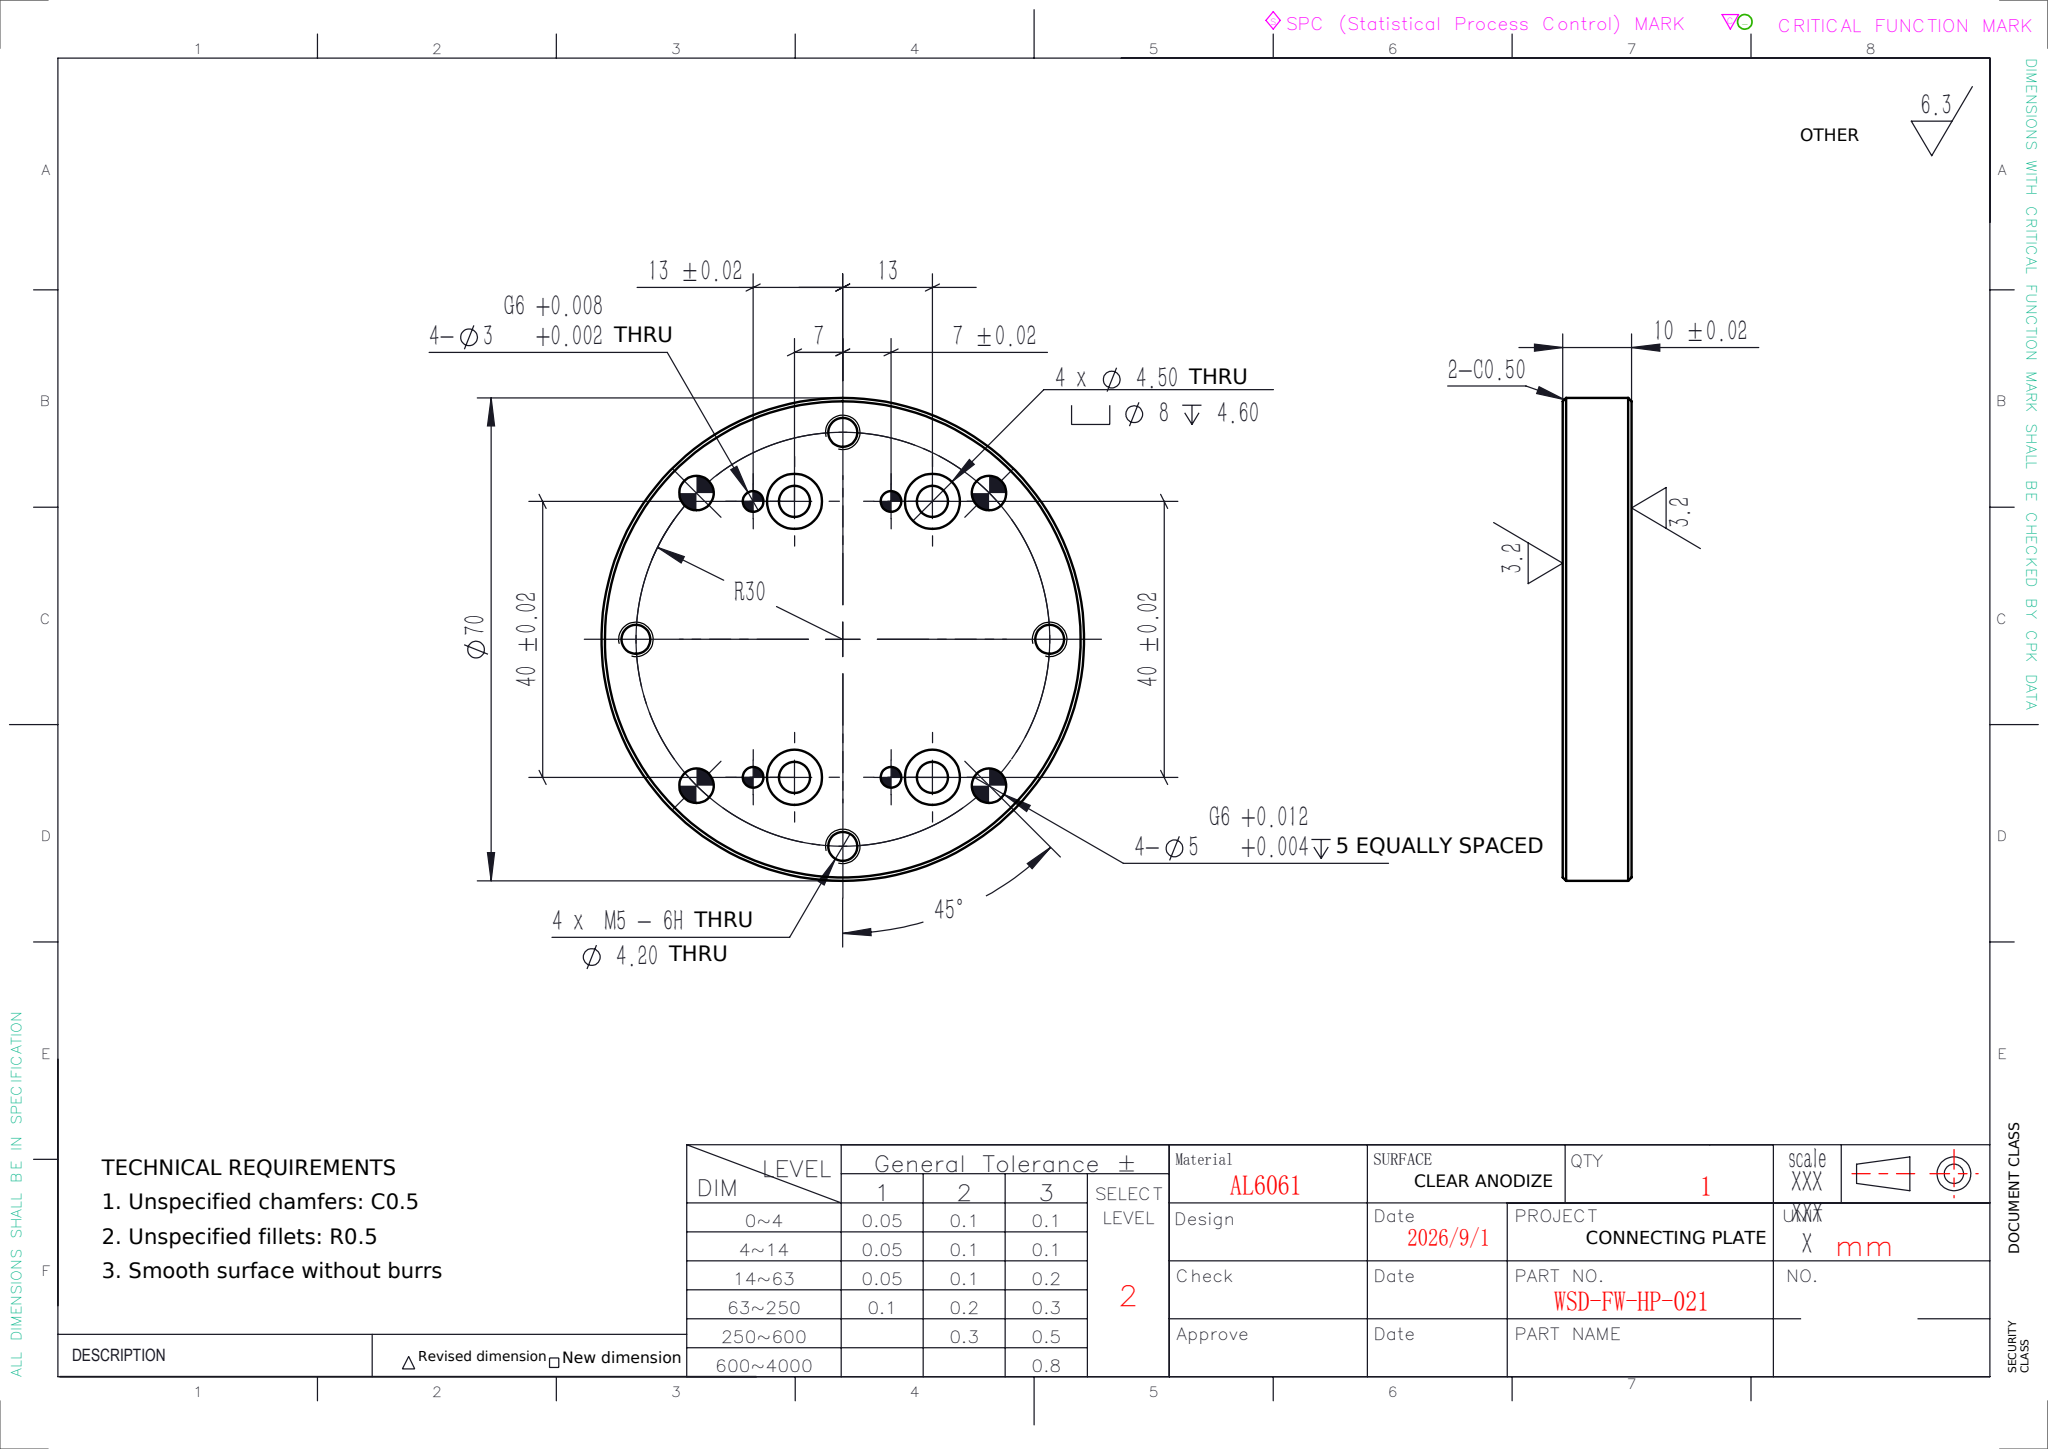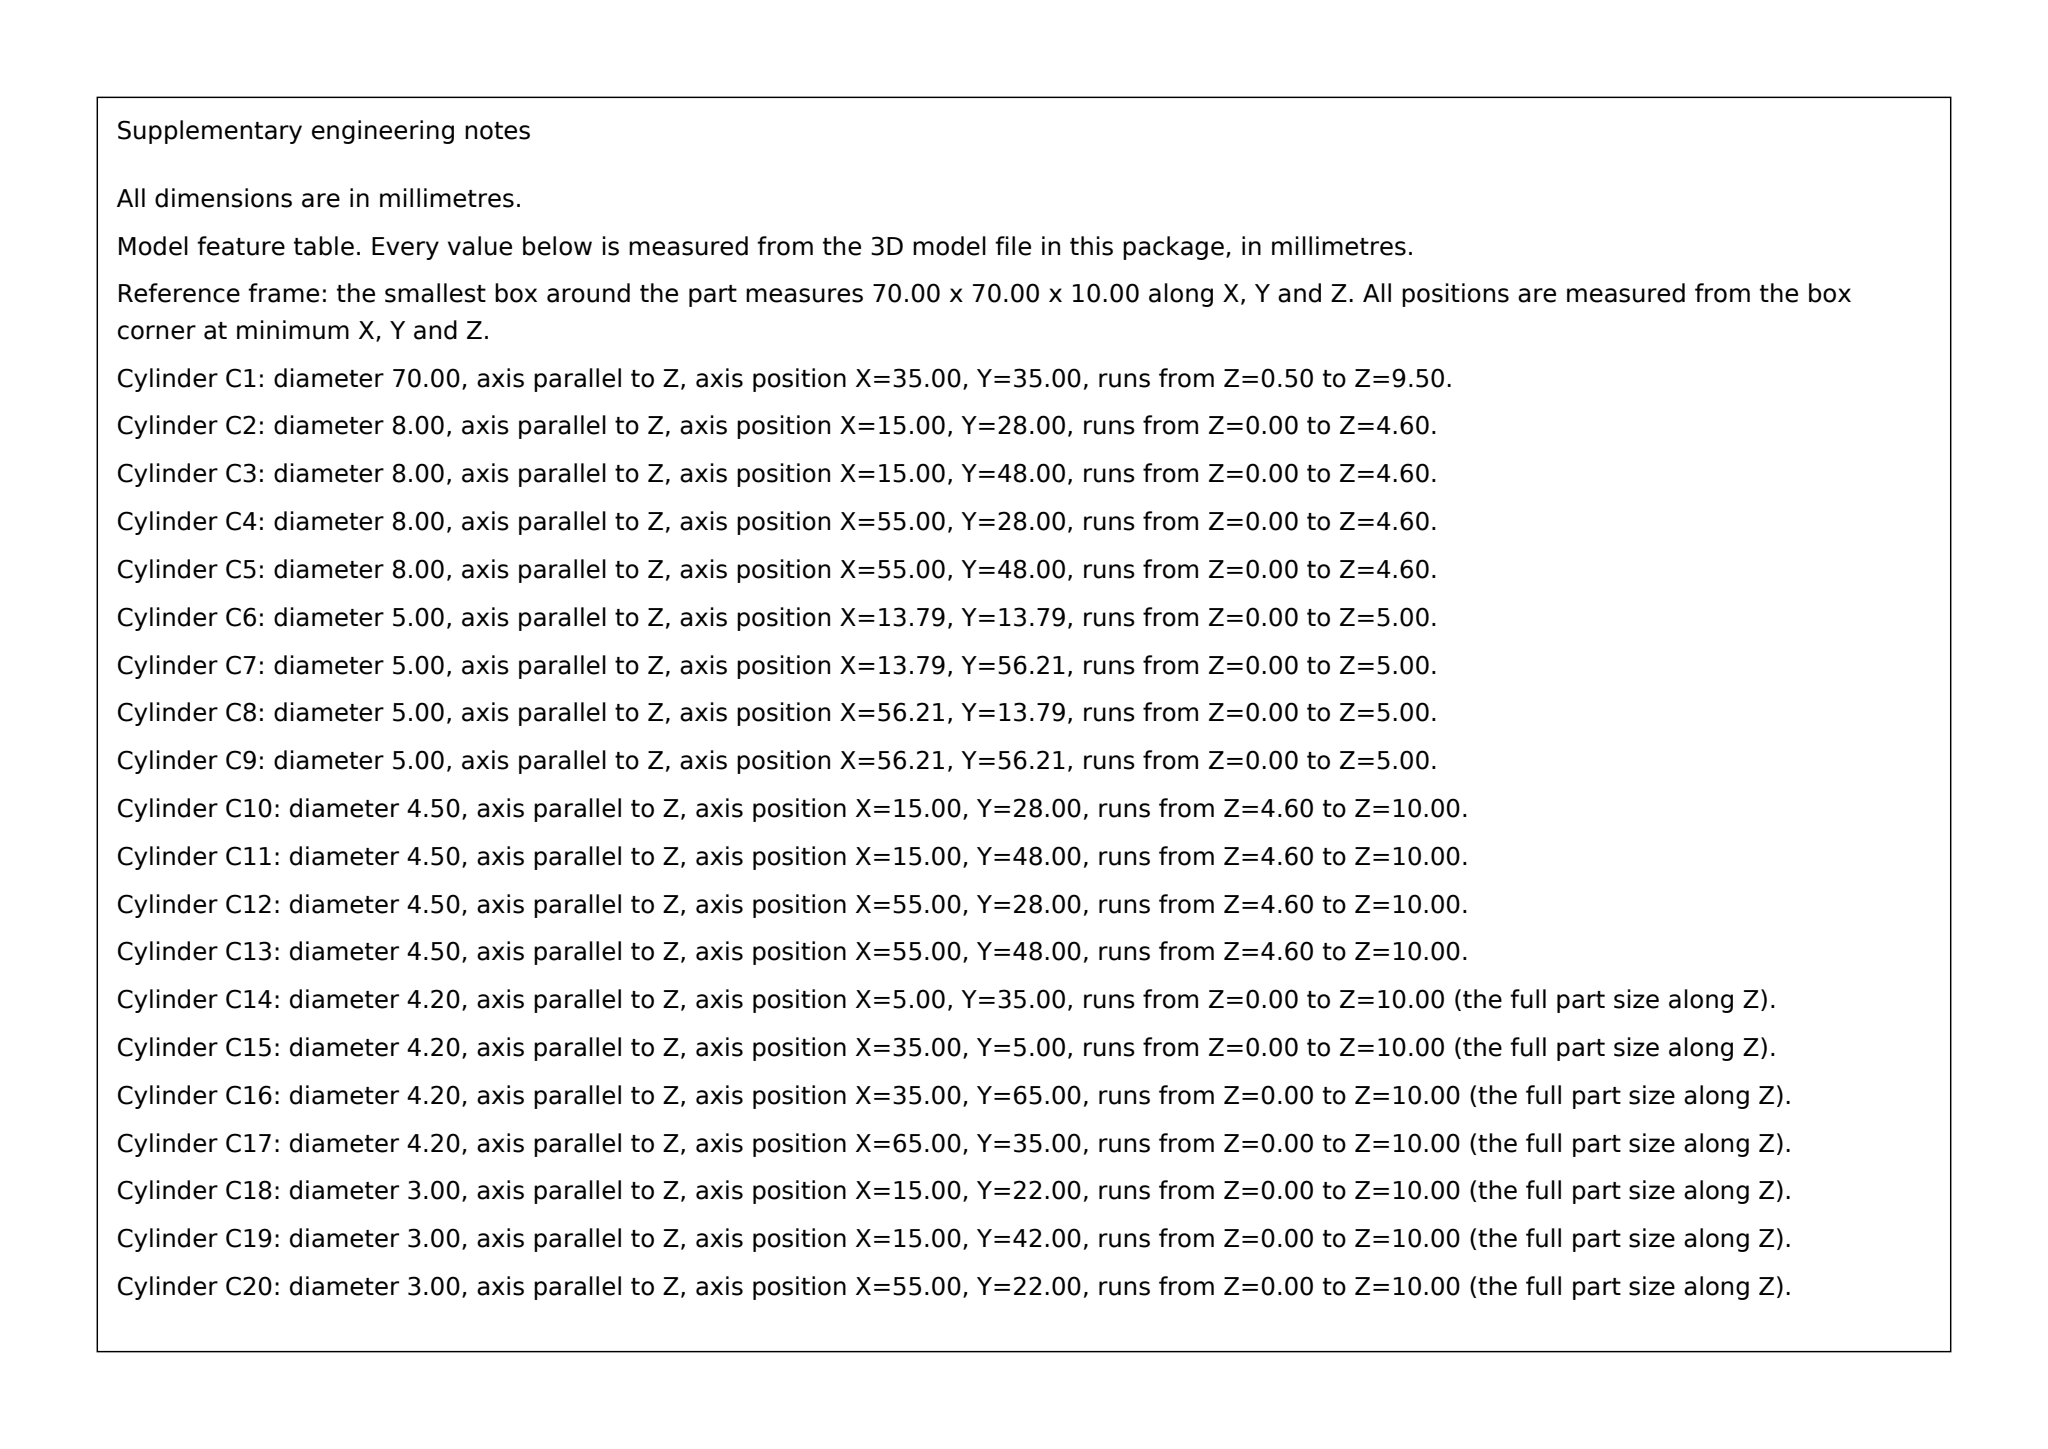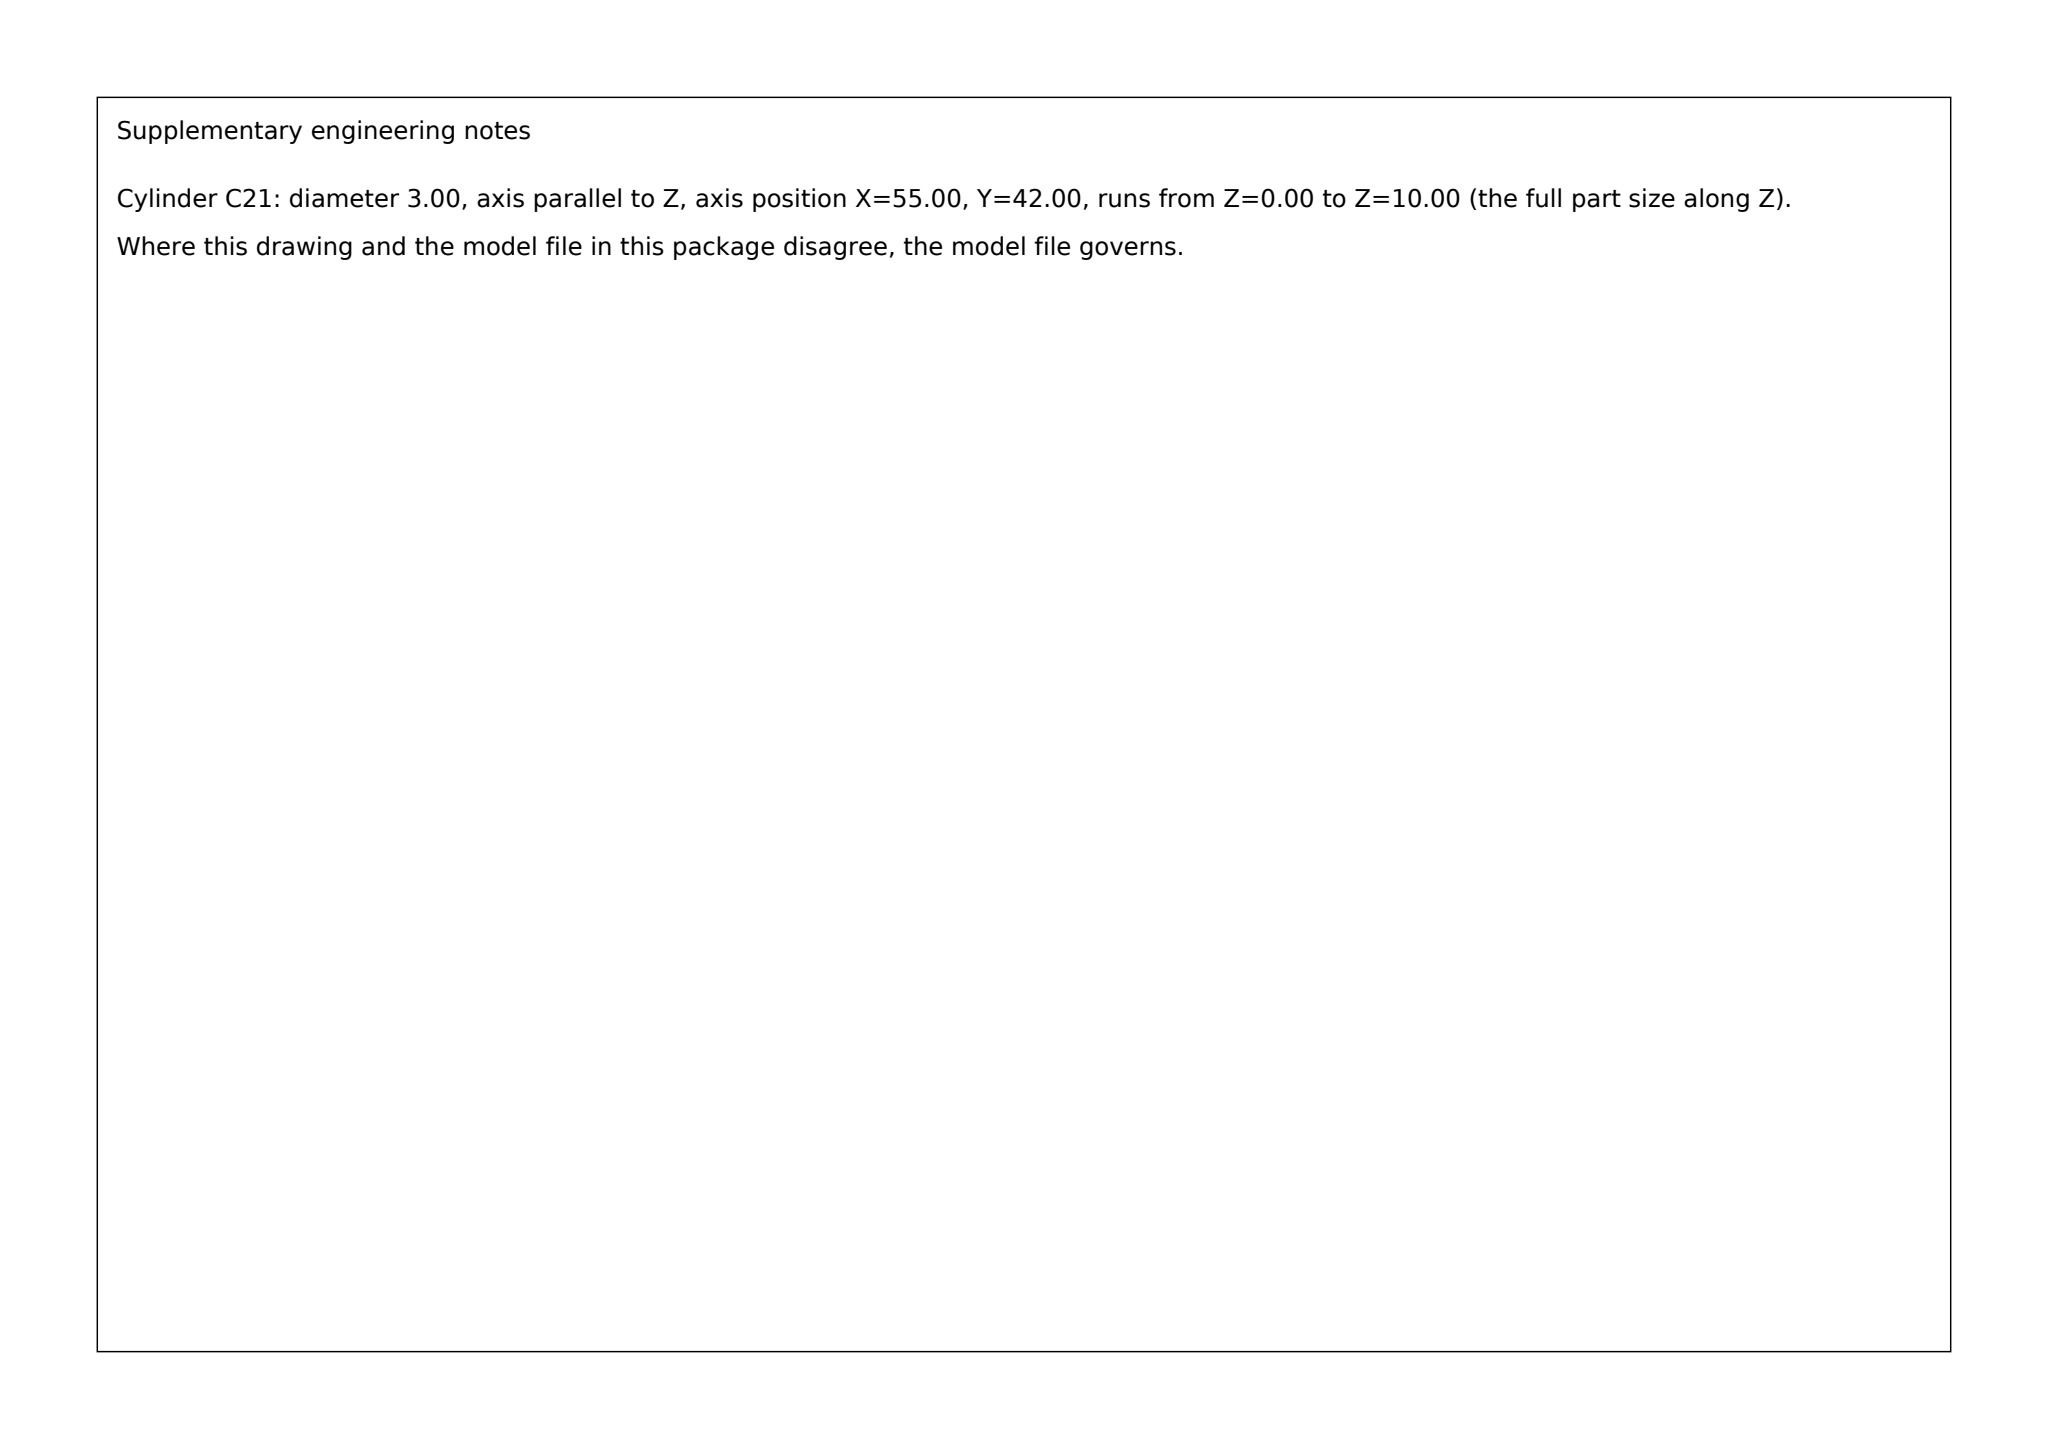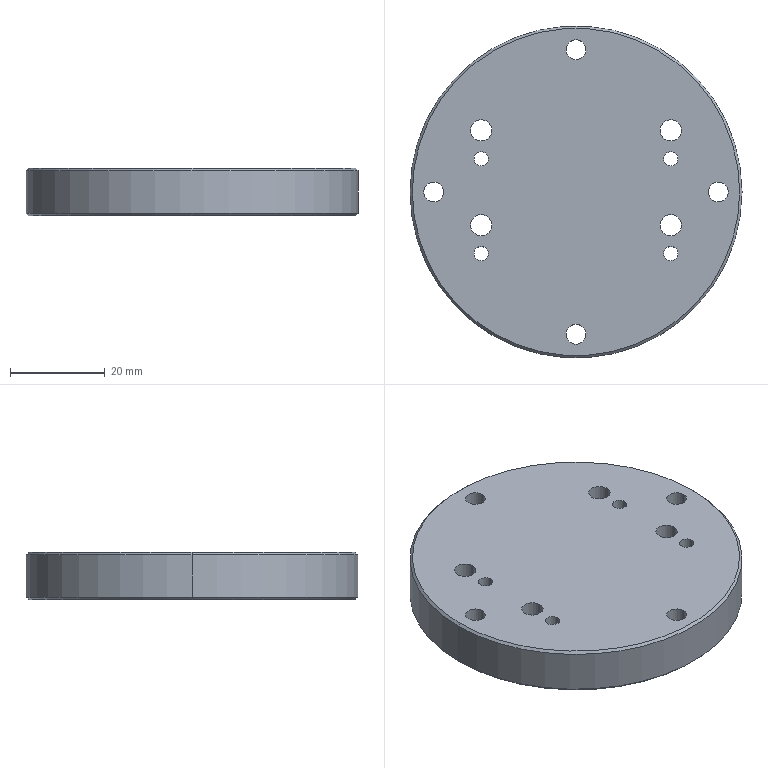Part | SolidWorks | mm | 1 solid | 56 faces | box 70 x 70 x 10 mm | volume 35932 mm3 | cylinder 42 | plane 10 | cone 4 | commonest cylinder face diameters 3 x8 5 x8 4.2 x8 8 x8 4.5 x8 70 x2
build123d program:
from build123d import *

# Parameters (mm, degrees)
SKETCH1_W                                         = 70
SKETCH1_H                                         = 70
BOSS_EXTRUDE1_DEPTH                               = 10
HOLE_SIZE_ACCORDING_TO_TYPE_0_OF_HEXA_D           = 4.5
HOLE_SIZE_ACCORDING_TO_TYPE_0_OF_HEXA_CBORE_D     = 8
HOLE_SIZE_ACCORDING_TO_TYPE_0_OF_HEXA_CBORE_DEPTH = 4.6
M5_TAPPED_HOLE1_D                                 = 4.2
SKETCH6_R                                         = 2.5
CUT_EXTRUDE1_DEPTH                                = 5
SKETCH7_R                                         = 1.5
CUT_EXTRUDE2_DEPTH                                = 51.498
CUT_EXTRUDE3_DEPTH                                = 51.498
CHAMFER1_SIZE                                     = 0.5


with BuildPart() as part:
    # Sketch1 → Boss-Extrude1 (new body)
    with BuildSketch(Plane.XY):
        Rectangle(SKETCH1_W, SKETCH1_H)
    extrude(amount=BOSS_EXTRUDE1_DEPTH)

    # Hole Size _ according to_ Type 0 of Hexa (through all)
    with Locations(Plane(origin=(0, 0, 0), x_dir=(-1, 0, 0), z_dir=(0, 0, -1))):
        with Locations((-20, 13), (-20, -7), (20, -7), (20, 13)):
            CounterBoreHole(HOLE_SIZE_ACCORDING_TO_TYPE_0_OF_HEXA_D / 2, HOLE_SIZE_ACCORDING_TO_TYPE_0_OF_HEXA_CBORE_D / 2, HOLE_SIZE_ACCORDING_TO_TYPE_0_OF_HEXA_CBORE_DEPTH)

    # M5 Tapped Hole1 (through all)
    with Locations(Plane(origin=(0, 0, 0), x_dir=(-1, 0, 0), z_dir=(0, 0, -1))):
        with Locations((0, 30), (-30, 0), (30, 0), (0, -30)):
            Hole(M5_TAPPED_HOLE1_D / 2)

    # Sketch6 → Cut-Extrude1 (cut)
    with BuildSketch(Plane(origin=(0, 0, 0), x_dir=(-1, 0, 0), z_dir=(0, 0, -1))):
        with Locations((21.213, 21.213)):
            Circle(SKETCH6_R)
        with Locations((-21.213, 21.213)):
            Circle(SKETCH6_R)
        with Locations((-21.213, -21.213)):
            Circle(SKETCH6_R)
        with Locations((21.213, -21.213)):
            Circle(SKETCH6_R)
    extrude(amount=-CUT_EXTRUDE1_DEPTH, mode=Mode.SUBTRACT)

    # Sketch7 → Cut-Extrude2 (cut, through all)
    with BuildSketch(Plane(origin=(0, 0, 0), x_dir=(-1, 0, 0), z_dir=(0, 0, -1))):
        with Locations((-20, 7)):
            Circle(SKETCH7_R)
        with Locations((-20, -13)):
            Circle(SKETCH7_R)
        with Locations(Location((20, -13, 0), (0, 0, 180))):
            Circle(SKETCH7_R)
        with Locations(Location((20, 7, 0), (0, 0, 180))):
            Circle(SKETCH7_R)
    extrude(amount=-CUT_EXTRUDE2_DEPTH, mode=Mode.SUBTRACT)

    # Sketch8 → Cut-Extrude3 (cut, through all)
    with BuildSketch(Plane(origin=(0, 0, 0), x_dir=(-1, 0, 0), z_dir=(0, 0, -1))):
        with BuildLine():
            Line((0, 35), (-35, 35))
            Line((-35, 35), (-35, 0))
            ThreePointArc((-35, 0), (-24.749, 24.749), (0, 35))
        make_face()
        with BuildLine():
            Line((35, 35), (0, 35))
            ThreePointArc((0, 35), (24.749, 24.749), (35, 0))
            Line((35, 0), (35, 35))
        make_face()
        with BuildLine():
            Line((35, -35), (35, 0))
            ThreePointArc((35, 0), (24.749, -24.749), (0, -35))
            Line((0, -35), (35, -35))
        make_face()
        with BuildLine():
            ThreePointArc((0, -35), (-24.749, -24.749), (-35, 0))
            Line((-35, 0), (-35, -35))
            Line((-35, -35), (0, -35))
        make_face()
    extrude(amount=-CUT_EXTRUDE3_DEPTH, mode=Mode.SUBTRACT)

    # Chamfer1
    chamfer1_edges = [part.edges().sort_by_distance(p)[0] for p in [
        (35, 0, 0),
        (35, 0, 10),
    ]]
    chamfer(chamfer1_edges, length=CHAMFER1_SIZE)


solid = part.part